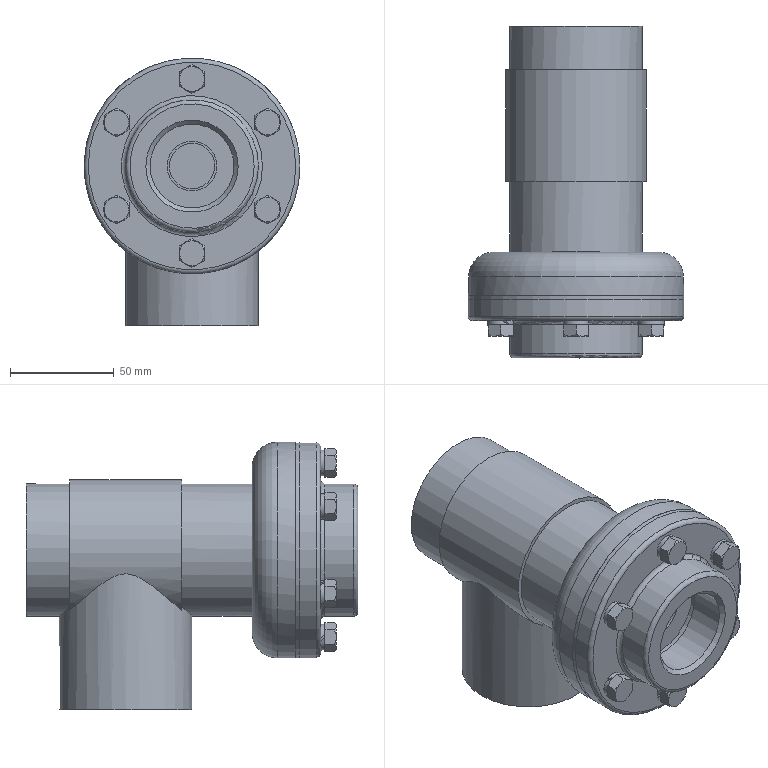Assembly | NX | mm | 28 component files | 28 solids | 457 faces | box 104 x 160 x 129 mm | volume 592072 mm3 | plane 227 | cylinder 121 | cone 87 | torus 17 | spline 5 | commonest cylinder face diameters 8 x16 9 x12 4 x8 42 x8 12.4 x6 8.2 x6 28 x5 64 x4
Bill of materials:
unnamed part 1 | 4 |  | Hex-head bolt-like part with a plain cylindrical shank and a small cross hole through the hex head.
unnamed part 2 | 1 |  | Pipe-fitting-like body: a flanged end on a straight cylindrical run, with a perpendicular cylindrical branch joined to it.
unnamed part 3 | 1 |  | Round flange with a cylindrical hub, a central through bore and six through holes on a bolt circle.
unnamed part 4 | 4 |  | Split ring of rectangular cross-section with one angled radial cut.
unnamed part 5 | 6 |  | Hex-head bolt-like part with a plain cylindrical shank.
unnamed part 6 | 1 |  | Thin flat annular disc with a large central opening and six holes on a bolt circle.
unnamed part 7 | 1 |  | Closed loop of thin round wire or rod, shaped like a rounded octagon, with one small gap.
unnamed part 8 | 6 |  | Split ring of rectangular cross-section with an angled cut and clearly offset ends.
unnamed part 9 | 1 |  | Hollow cylindrical housing with a reduced-diameter stepped end carrying slots/flats and a chamfered end disc.
unnamed part 10 | 1 |  | Helical coil of round wire with closed, flattened end coils.
unnamed part 11 | 1 |  | Flat circular plate with a central bore, four holes on a bolt circle and two raised lugs on one face.
unnamed part 12 | 1 |  | Plain solid cylinder (short round disc or slug).
Mates:
1. fix | valve_body 1 component
2. touch align | gasket 1 face | valve_body 1 face
3. concentric | gasket 1 edge | valve_body 1 edge
4. touch align | end_cap 1 face | gasket 1 face
5. concentric | end_cap 1 edge | gasket 1 edge
6. touch align | valve_disc 1 face | valve_body 1 face
7. touch align | valve_disc 1 face | valve_body 1 face
8. touch align | cover 1 face | valve_disc 1 face
9. concentric | cover 1 edge | valve_disc 1 edge
10. concentric | spring 1 edge | cup 1 edge
11. concentric | cup 1 edge | cover 1 edge
12. concentric | spring_washer_4 4 edge | bolt_M4x10 4 edge
13. bond | valve_body 1 component | assembly component
14. bond | spring_washer_4 4 component | assembly component
15. bond | bolt_M4x10 4 component | assembly component
16. bond | spring_washer_4 3 component | assembly component
17. bond | bolt_M4x10 3 component | assembly component
18. bond | spring_washer_4 2 component | assembly component
19. bond | bolt_M4x10 2 component | assembly component
20. bond | spring_washer_4 1 component | assembly component
21. bond | bolt_M4x10 1 component | assembly component
22. circular | assembly datumaxis | assembly cartesiancoordinatesystem | assembly cartesiancoordinatesystem | assembly cartesiancoordinatesystem | assembly cartesiancoordinatesystem
23. circular | assembly datumaxis | assembly cartesiancoordinatesystem | assembly cartesiancoordinatesystem | assembly cartesiancoordinatesystem | assembly cartesiancoordinatesystem
24. concentric | spring_washer_4 4 edge | cover 1 edge
25. touch align | steel_wire 1 face | bolt_M4x10 4 face
26. touch align | steel_wire 1 face | bolt_M4x10 3 face
27. concentric | spring_washer_8 6 edge | bolt_M8x20 6 edge
28. concentric | spring_washer_8 6 edge | end_cap 1 edge
29. bond | end_cap 1 component | assembly component
30. bond | spring_washer_8 6 component | assembly component
31. bond | bolt_M8x20 6 component | assembly component
32. bond | spring_washer_8 5 component | assembly component
33. bond | bolt_M8x20 5 component | assembly component
34. bond | spring_washer_8 4 component | assembly component
35. bond | bolt_M8x20 4 component | assembly component
36. bond | spring_washer_8 3 component | assembly component
37. bond | bolt_M8x20 3 component | assembly component
38. circular | assembly datumaxis | assembly cartesiancoordinatesystem | assembly cartesiancoordinatesystem | assembly cartesiancoordinatesystem | assembly cartesiancoordinatesystem | assembly cartesiancoordinatesystem | assembly cartesiancoordinatesystem
39. circular | assembly datumaxis | assembly cartesiancoordinatesystem | assembly cartesiancoordinatesystem | assembly cartesiancoordinatesystem | assembly cartesiancoordinatesystem | assembly cartesiancoordinatesystem | assembly cartesiancoordinatesystem
40. bond | spring_washer_8 2 component | assembly component
41. bond | bolt_M8x20 2 component | assembly component
42. bond | spring_washer_8 1 component | assembly component
43. bond | bolt_M8x20 1 component | assembly component